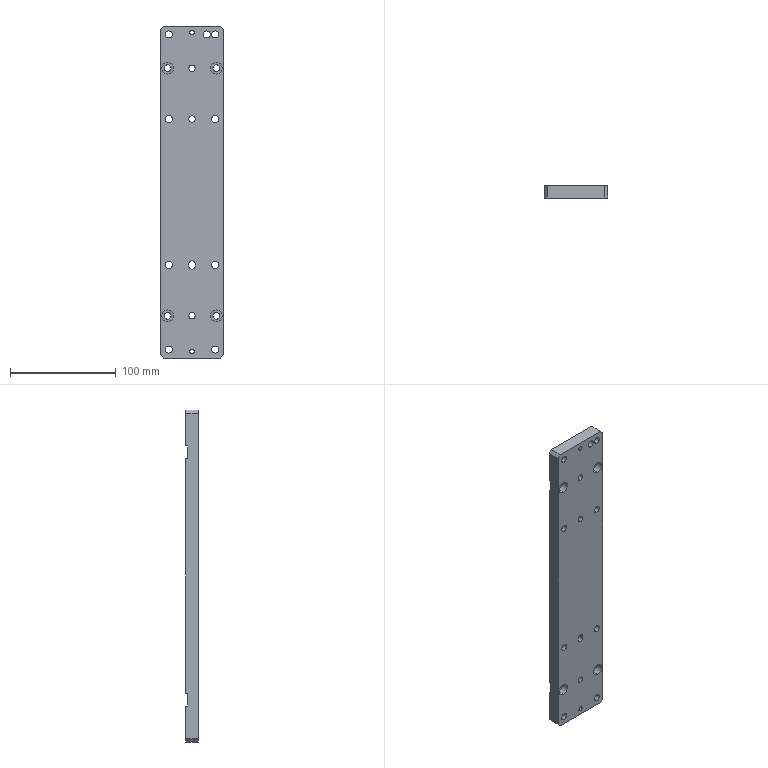Component | SolidWorks | 01-1111-1 | 1 solid | 87 faces | box 60 x 12 x 314 mm | volume 212923 mm3 | cylinder 47 | plane 40 | commonest cylinder face diameters 6.6 x26 6 x9 11 x8 4.2 x4
build123d program:
from build123d import *

# Parameters (mm, degrees)
SKETCH1_2_W                                    = 60
SKETCH1_2_H                                    = 314
BOSS_EXTRUDE1_DEPTH                            = 12
SKETCH4_W                                      = 60
SKETCH4_H                                      = 12
CUT_EXTRUDE4_DEPTH                             = 2
M6_HEX_SOCKET_HEAD_CAP_SCREW_CBORE1_AT_2_COUNT = 2
M6_HEX_SOCKET_HEAD_CAP_SCREW_CBORE1_AT_2_PITCH = 46
M6_CLEARANCE_HOLE1_D                           = 6.6
LPATTERN1_COUNT                                = 2
LPATTERN1_PITCH                                = 80
SIZE_MM_DOWEL_PIN_HOLE_2_D                     = 6
MIRROR2_COPY_1_D                               = 6.6
CUT_EXTRUDE5_DEPTH                             = 161.29
CHAMFER1_SIZE                                  = 3
M5_TAPPED_HOLE1_D                              = 4.2
M6_CLEARANCE_HOLE2_D                           = 6.6
RELIEF_09_BRACKET_DEPTH                        = 9.2


with BuildPart() as part:
    # Sketch1_2 → Boss-Extrude1 (new body)
    with BuildSketch(Plane(origin=(0, 0, 0), x_dir=(1, 0, 0), z_dir=(0, 1, 0))):
        Rectangle(SKETCH1_2_W, SKETCH1_2_H)
    extrude(amount=BOSS_EXTRUDE1_DEPTH)

    # Sketch4 → Cut-Extrude4 (cut)
    with BuildSketch(Plane(origin=(0, 12, 0), x_dir=(1, 0, 0), z_dir=(0, 1, 0))):
        with Locations((0, 117)):
            Rectangle(SKETCH4_W, SKETCH4_H)
        with Locations((0, -117)):
            Rectangle(SKETCH4_W, SKETCH4_H)
    extrude(amount=-CUT_EXTRUDE4_DEPTH, mode=Mode.SUBTRACT)

    # Sketch6 → M6 Hex Socket Head Cap Screw CBORE1 (revolve, cut)
    with BuildSketch(Plane(origin=(23, 0, -117), x_dir=(0, 0, -1), z_dir=(1, 0, 0))):
        Polygon((0, 0), (0, 18.983), (3.3, 17), (3.3, 6.4), (5.5, 6.4), (5.5, 0), align=None)
    m6_hex_socket_head_cap_screw_cbore1 = revolve(axis=Axis((23, -6.35, -117), (0, 1, 0)), mode=Mode.SUBTRACT)

    # M6 Hex Socket Head Cap Screw CBORE1 at 2: M6 Hex Socket Head Cap Screw CBORE1 ×2
    with Locations(*[(-i * M6_HEX_SOCKET_HEAD_CAP_SCREW_CBORE1_AT_2_PITCH, 0, 0) for i in range(1, M6_HEX_SOCKET_HEAD_CAP_SCREW_CBORE1_AT_2_COUNT)]):
        add(m6_hex_socket_head_cap_screw_cbore1, mode=Mode.SUBTRACT)

    # Sketch8 → Size mm Dowel Pin Hole 1 (revolve, cut)
    with BuildSketch(Plane(origin=(0, 0, -117), x_dir=(0, 0, -1), z_dir=(1, 0, 0))):
        Polygon((0, 0), (0, 18.803), (3, 17), (3, 0), align=None)
    size_mm_dowel_pin_hole_1 = revolve(axis=Axis((0, -6.35, -117), (0, 1, 0)), mode=Mode.SUBTRACT)

    # Mirror1: M6 Hex Socket Head Cap Screw CBORE1, Size mm Dowel Pin Hole 1 across plane
    add(m6_hex_socket_head_cap_screw_cbore1.mirror(Plane.XY), mode=Mode.SUBTRACT)
    add(size_mm_dowel_pin_hole_1.mirror(Plane.XY), mode=Mode.SUBTRACT)

    # Mirror1 copy 1 sketch → Mirror1 copy 1 (revolve, cut)
    with BuildSketch(Plane(origin=(-23, 0, 117), x_dir=(0, 0, 1), z_dir=(1, 0, 0))):
        Polygon((0, 0), (0, -18.983), (3.3, -17), (3.3, -6.4), (5.5, -6.4), (5.5, 0), align=None)
    revolve(axis=Axis((-23, -6.35, 117), (0, -1, 0)), mode=Mode.SUBTRACT)

    # M6 Clearance Hole1 (through all)
    with Locations(Plane(origin=(0, 12, 0), x_dir=(1, 0, 0), z_dir=(0, 1, 0))):
        with Locations((22, 149), (-22, 149)):
            m6_clearance_hole1 = Hole(M6_CLEARANCE_HOLE1_D / 2)

    # LPattern1: M6 Clearance Hole1 ×2
    with Locations(*[(0, 0, i * LPATTERN1_PITCH) for i in range(1, LPATTERN1_COUNT)]):
        add(m6_clearance_hole1, mode=Mode.SUBTRACT)

    # Size mm Dowel Pin Hole 2 (through all)
    with Locations(Plane(origin=(0, 12, 0), x_dir=(1, 0, 0), z_dir=(0, 1, 0))):
        with Locations((0, 69)):
            size_mm_dowel_pin_hole_2 = Hole(SIZE_MM_DOWEL_PIN_HOLE_2_D / 2)

    # Mirror2: M6 Clearance Hole1, Size mm Dowel Pin Hole 2 across plane
    add(m6_clearance_hole1.mirror(Plane.XY), mode=Mode.SUBTRACT)
    add(size_mm_dowel_pin_hole_2.mirror(Plane.XY), mode=Mode.SUBTRACT)

    # Mirror2 copy 1 (through all)
    with Locations(Plane(origin=(0, 12, -80), x_dir=(1, 0, 0), z_dir=(0, 1, 0))):
        with Locations((22, -149), (-22, -149)):
            Hole(MIRROR2_COPY_1_D / 2)

    # Sketch14 → Cut-Extrude5 (cut, through all)
    with BuildSketch(Plane(origin=(0, 12, 0), x_dir=(1, 0, 0), z_dir=(0, 1, 0))):
        with BuildLine():
            Line((3, 70), (3, 68))
            ThreePointArc((3, 68), (0, 65), (-3, 68))
            Line((-3, 68), (-3, 70))
            ThreePointArc((-3, 70), (0, 73), (3, 70))
        make_face()
    extrude(amount=-CUT_EXTRUDE5_DEPTH, mode=Mode.SUBTRACT)

    # Chamfer1
    chamfer1_edges = [part.edges().sort_by_distance(p)[0] for p in [
        (30, 6, 157),
        (-30, 6, 157),
        (-30, 6, -157),
        (30, 6, -157),
    ]]
    chamfer(chamfer1_edges, length=CHAMFER1_SIZE)

    # M5 Tapped Hole1 (through all)
    with Locations(Plane(origin=(0, 12, 0), x_dir=(1, 0, 0), z_dir=(0, 1, 0))):
        with Locations((0, -151)):
            m5_tapped_hole1 = Hole(M5_TAPPED_HOLE1_D / 2)

    # Mirror3: M5 Tapped Hole1 across plane
    add(m5_tapped_hole1.mirror(Plane.XY), mode=Mode.SUBTRACT)

    # M6 Clearance Hole2 (through all)
    with Locations(Plane(origin=(0, 12, 0), x_dir=(1, 0, 0), z_dir=(0, 1, 0))):
        with Locations((14, -149)):
            Hole(M6_CLEARANCE_HOLE2_D / 2)

    # Sketch1 → Relief-09-bracket (cut, symmetric)
    with BuildSketch(Plane(origin=(0, 12, 0), x_dir=(1, 0, 0), z_dir=(0, 1, 0))):
        Polygon((-14.2, 143.2), (-11.5, 143.2), (-11.5, 125.2), (6.2, 125.2), (6.2, 123), (-14.2, 123), align=None)
        Polygon((-14.2, -123), (6.2, -123), (6.2, -125.2), (-11.5, -125.2), (-11.5, -143.2), (-14.2, -143.2), align=None)
    extrude(amount=RELIEF_09_BRACKET_DEPTH, both=True, mode=Mode.SUBTRACT)


solid = part.part

# Placed as in the assembly
solid = solid.moved(Location((-135.072, 396.224, 1393.056), (0, 0, 0)))